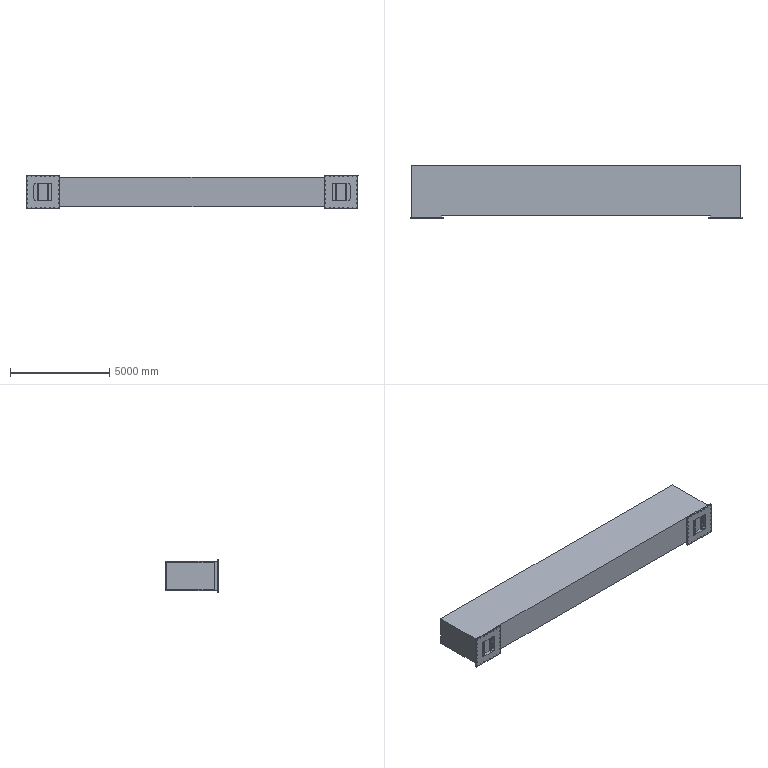Component | SolidWorks | LowerCrossbeam-3 | 1 solid | 340 faces | volume 9493103476 mm3 | plane 172 | cylinder 168 | commonest cylinder face diameters 40 x112 200 x56